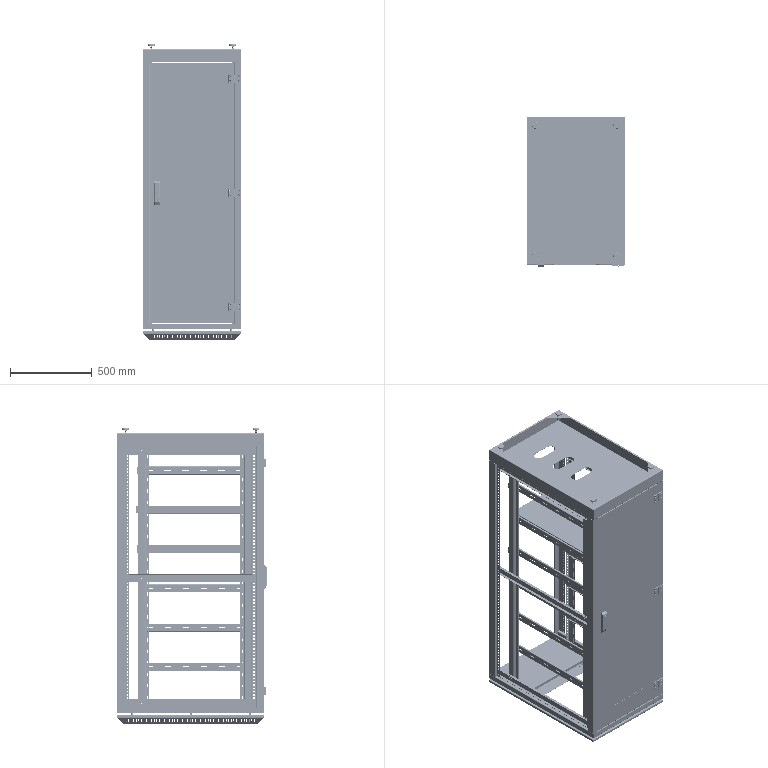Assembly | SolidWorks | mm | 69 component files | 69 solids | 8213 faces | box 600 x 916 x 1803.5 mm | volume 13058745 mm3 | plane 5185 | cylinder 2836 | spline 140 | cone 52 | commonest cylinder face diameters 3 x780 6 x617 5 x588 7 x278 12 x200 2 x165 10 x51 6.8 x40
Bill of materials:
ChassisWheel | 4 |  | Screw-like part: a large, flat, disc-shaped head with chamfered edges on a shorter, smaller-diameter shank that is threaded along most of its length.
Column | 3 |  | Long, slender bent sheet profile whose cross-section has several right-angle bends with rounded corners, forming a stepped, offset channel shape. A row of small perforations runs along its length.
Drawer | 1 |  | Shallow rectangular tray or cover panel: a flat face with short flanges folded down on all four edges.
Handle | 1 |  | Long bent sheet profile: a vertical wall, a flat top, an angled sloping section, and a short downturned lip, all with rounded bends.
828LockHead | 1 |  | Compact multi-feature body that looks like a latch or handle mechanism: an elongated front housing with a recessed face, a stepped rear body, a rectangular window, and a pin with a flanged head sticking out sideways.
LockRod | 2 |  | Pin with a flat tab: a flat, rounded-end tab with two through holes on top of a cylindrical rod with a conical tip.
LowerPullRod | 1 |  | Narrow flat strip with two joggle (offset) bends, giving a stepped profile, and two round holes near its rounded upper end.
UpperPullRod | 1 |  | Narrow flat strip with a single joggle bend: a long plain upper section and an offset lower section with a rounded end and two round holes.
BentPlate | 2 |  | Very long, slender U-channel with rounded bends and small holes spaced along its length.
GlassDoor | 1 |  | Thin flat rectangular frame panel with a large rounded-rectangle central cutout, two small rectangular cutouts in one side member, and small holes along the opposite edge.
ShortBentPlate_2 | 2 |  | Long bent sheet bracket with a stepped Z/hat-like section: a vertical web with three obround slots, a bottom flange, and an offset top flange that is shorter than the web.
ShortBentPlate | 2 |  | Straight C-channel with rounded bends and three small round holes in the web.
TemperedGlass5mm | 1 |  | Thin, plain rectangular flat plate, long and narrow, with no visible holes or cutouts.
GussetPlate | 4 |  | Thin flat plate shaped as a right-angle triangle with two equal legs and one circular through-hole near the right-angle corner.
Nut | 4 |  | Hexagonal prism with a central bore that has internal thread grooves (nut-like). One end has curved chamfered edges on the corners.
HexRod | 6 |  | Long, slender hexagonal bar with chamfered end corners and a threaded-looking axial hole at the visible end (standoff-like).
InnerColumn | 4 |  | Long formed sheet-metal profile with a stepped, multi-bend cross-section (a flange, a step, a long web and a return flange) with rounded bends, perforated along its length with regularly spaced slots and holes.
LeftColumn | 1 |  | Long formed sheet-metal profile with a complex stepped cross-section (outer flange, step, deep U-shaped section and opposite flange), rounded bends, small holes along one flange and notched ends.
LowerSeat | 1 |  | Shallow rectangular tray: a flat base with four upturned perimeter walls, three parallel obround slots in the base and small holes near the side edges.
OuterDoorHinge3 | 3 |  | Hinge-leaf-shaped plate: a flat rectangular leaf with two countersunk through-holes, an angled edge on one side, and three cylindrical knuckles with an axial bore along the opposite edge.
OuterHinge4 | 3 |  | Hinge-leaf-shaped plate: a flat rectangular leaf with two countersunk through-holes, an angled edge on one side, and two cylindrical knuckles with an axial bore along the opposite edge.
RailMountingBeam | 12 |  | Long, slender formed sheet-metal bracket/rail: a narrow web with six evenly spaced elongated slots, edge flanges, and a bent end tab at each end with two obround slots.
SideFixingBeam | 6 |  | Long straight bar with a rectangular, round-cornered cross-section (likely formed sheet), with one elongated slot near each end on one face and one small round hole near each end on an adjacent face.
TopCover | 1 |  | Rectangular sheet-metal panel/frame with a large rectangular cutout, inclined perimeter flanges with rows of narrow ventilation-style slots, and several small holes in the flat area.
UpperSeat2 | 1 |  | Thin, flat, U-shaped (forked) plate that looks like formed sheet metal. A solid rectangular region joins two long parallel legs, with a large rectangular open slot between them. Shallow flanges are bent down along the outer edges, and the face has small round through-holes.
UpperSill | 1 |  | Long, narrow, open-bottomed channel that looks like formed sheet metal. It has a flat top web and bent side walls with return lips at the bottom. One end is closed by a flange with a row of five evenly spaced round holes.
Mates:
1. coincident | LowerSeat-1 face at (-487.577, 386.781, 78) dir (1, 0, 0) | GussetPlateAssembly-1/GussetPlate-1 face at (-487.577, 276.923, 78) dir (-1, 0, 0)
2. coincident | LowerSeat-1 face at (98.282, 376.923, 78) dir (0, -1, 0) | GussetPlateAssembly-1/GussetPlate-1 face at (-487.577, 376.923, 78) dir (0, 1, 0)
3. coincident | LowerSeat-1 face at (-497.435, 386.923, 78) dir (0, 0, 1) | GussetPlateAssembly-1/GussetPlate-1 face at (-387.577, 376.923, 78) dir (0, 0, 1)
4. coincident | LowerSeat-1 face at (98.282, 376.923, 78) dir (0, -1, 0) | GussetPlateAssembly-2/GussetPlate-1 face at (-11.577, 376.923, 78) dir (0, 1, 0)
5. coincident | LowerSeat-1 face at (88.423, -508.936, 78) dir (-1, 0, 0) | GussetPlateAssembly-2/GussetPlate-1 face at (88.423, 376.923, 78) dir (1, 0, 0)
6. coincident | LowerSeat-1 face at (-497.435, 386.923, 78) dir (0, 0, 1) | GussetPlateAssembly-2/GussetPlate-1 face at (88.423, 276.923, 78) dir (0, 0, 1)
7. coincident | LowerSeat-1 face at (-497.435, -499.077, 78) dir (0, 1, 0) | GussetPlateAssembly-4/GussetPlate-1 face at (88.423, -499.077, 78) dir (0, -1, 0)
8. coincident | LowerSeat-1 face at (88.423, -508.936, 78) dir (-1, 0, 0) | GussetPlateAssembly-4/GussetPlate-1 face at (88.423, -399.077, 78) dir (1, 0, 0)
9. coincident | LowerSeat-1 face at (98.423, 386.781, 78) dir (0, 0, 1) | GussetPlateAssembly-4/GussetPlate-1 face at (-11.577, -499.077, 78) dir (0, 0, 1)
10. coincident | LowerSeat-1 face at (-487.577, 386.781, 78) dir (1, 0, 0) | GussetPlateAssembly-3/GussetPlate-1 face at (-487.577, -499.077, 78) dir (-1, 0, 0)
11. coincident | LowerSeat-1 face at (-497.435, -499.077, 78) dir (0, 1, 0) | GussetPlateAssembly-3/GussetPlate-1 face at (-387.577, -499.077, 78) dir (0, -1, 0)
12. coincident | LowerSeat-1 face at (98.282, -509.077, 78) dir (0, 0, 1) | GussetPlateAssembly-3/GussetPlate-1 face at (-487.577, -399.077, 78) dir (0, 0, 1)
13. coincident | LowerSeat-1 face at (-499.577, -511.077, 0) dir (-1, 0, 0) | Column-2 face at (-499.577, -461.077, -2) dir (-1, 0, 0)
14. coincident | LowerSeat-1 face at (-499.577, -511.077, 78) dir (0, -1, 0) | Column-2 face at (-499.577, -511.077, -2) dir (0, -1, 0)
15. coincident | LowerSeat-1 face at (100.423, -511.077, -2) dir (0, 0, -1) | Column-2 face at (-496.577, -509.077, -2) dir (0, 0, 1)
16. coincident | LowerSeat-1 face at (100.423, 388.923, 78) dir (0, 1, 0) | Column-3 face at (-499.577, 388.923, -1597) dir (0, 1, 0)
17. coincident | LowerSeat-1 face at (-499.577, -511.077, 0) dir (-1, 0, 0) | Column-3 face at (-499.577, 338.923, -1597) dir (-1, 0, 0)
18. coincident | LowerSeat-1 face at (100.423, -511.077, -2) dir (0, 0, -1) | Column-3 face at (-496.577, 340.923, -2) dir (0, 0, 1)
19. coincident | LowerSeat-1 face at (100.423, 388.923, 78) dir (0, 1, 0) | Column-4 face at (100.423, 388.923, -2) dir (0, 1, 0)
20. coincident | LowerSeat-1 face at (100.423, -511.077, 78) dir (1, 0, 0) | Column-4 face at (100.423, 338.923, -2) dir (1, 0, 0)
21. coincident | LowerSeat-1 face at (100.423, -511.077, -2) dir (0, 0, -1) | Column-4 face at (62.423, 385.923, -2) dir (0, 0, 1)
22. coincident | Column-3 face at (-499.577, 388.923, -1597) dir (0, 1, 0) | UpperSeatAssembly-1/UpperSeat2-1 face at (100.423, 388.923, -1599) dir (0, 1, 0)
23. coincident | Column-3 face at (-499.577, 338.923, -1597) dir (-1, 0, 0) | UpperSeatAssembly-1/UpperSeat2-1 face at (-499.577, 388.923, -1599) dir (-1, 0, 0)
24. coincident | Column-3 face at (-496.577, 386.923, -1597) dir (0, 0, -1) | UpperSeatAssembly-1/UpperSeat2-1 face at (100.423, -511.077, -1597) dir (0, 0, 1)
25. coincident | LowerSeat-1 face at (100.423, -511.077, -2) dir (0, 0, -1) | SideFixingBeam-1 face at (-479.577, -488.077, -2) dir (0, 0, 1)
26. coincident | Column-3 face at (-479.577, 315.923, -1597) dir (1, 0, 0) | SideFixingBeam-1 face at (-479.577, 361.923, -2) dir (-1, 0, 0)
27. coincident | Column-3 face at (-459.577, 361.923, -1597) dir (0, -1, 0) | SideFixingBeam-1 face at (-479.577, 361.923, -2) dir (0, 1, 0)
28. coincident | LowerSeat-1 face at (100.423, -511.077, -2) dir (0, 0, -1) | SideFixingBeam-2 face at (80.423, 361.923, -2) dir (0, 0, 1)
29. coincident | Column-4 face at (62.423, 388.923, -2) dir (1, 0, 0) | SideFixingBeam-2 face at (62.423, 361.923, -2) dir (-1, 0, 0)
30. coincident | Column-4 face at (60.423, 361.923, -2) dir (0, -1, 0) | SideFixingBeam-2 face at (80.423, 361.923, -52) dir (0, 1, 0)
31. coincident | Column-4 face at (62.423, 388.923, -2) dir (1, 0, 0) | SideFixingBeam-3 face at (62.423, 361.923, -1547) dir (-1, 0, 0)
32. coincident | UpperSeatAssembly-1/UpperSeat2-1 face at (100.423, -511.077, -1597) dir (0, 0, 1) | SideFixingBeam-3 face at (80.423, -488.077, -1597) dir (0, 0, -1)
33. coincident | Column-4 face at (60.423, 361.923, -2) dir (0, -1, 0) | SideFixingBeam-3 face at (80.423, 361.923, -1597) dir (0, 1, 0)
34. coincident | Column-3 face at (-461.577, 388.923, -1597) dir (-1, 0, 0) | SideFixingBeam-5 face at (-461.577, 361.923, -1597) dir (1, 0, 0)
35. coincident | UpperSeatAssembly-1/UpperSeat2-1 face at (100.423, -511.077, -1597) dir (0, 0, 1) | SideFixingBeam-5 face at (-479.577, 361.923, -1597) dir (0, 0, -1)
36. coincident | Column-3 face at (-459.577, 361.923, -1597) dir (0, -1, 0) | SideFixingBeam-5 face at (-479.577, 361.923, -1547) dir (0, 1, 0)
37. coincident | Column-4 face at (60.423, 361.923, -2) dir (0, -1, 0) | SideFixingBeam-6 face at (80.423, 361.923, -832) dir (0, 1, 0)
38. coincident | Column-3 face at (-461.577, 388.923, -1597) dir (-1, 0, 0) | SideFixingBeam-7 face at (-461.577, 361.923, -832) dir (1, 0, 0)
39. coincident | Column-3 face at (-459.577, 361.923, -1597) dir (0, -1, 0) | SideFixingBeam-7 face at (-479.577, 361.923, -782) dir (0, 1, 0)
40. coincident | SideFixingBeam-1 face at (-461.577, 361.923, -52) dir (1, 0, 0) | InnerColumn-1 face at (-461.577, -388.077, -4.5) dir (-1, 0, 0)
41. distance | InnerColumn-1 face at (-461.577, -433.077, -4.5) dir (0, -1, 0) | LowerSeat-1 face at (-499.577, -511.077, 78) dir (0, -1, 0)
42. coincident | SideFixingBeam-2 face at (62.423, 361.923, -2) dir (-1, 0, 0) | InnerColumn-2 face at (62.423, -388.077, -1594.5) dir (1, 0, 0)
43. distance | InnerColumn-2 face at (62.423, -433.077, -1594.5) dir (0, -1, 0) | LowerSeat-1 face at (-499.577, -511.077, 78) dir (0, -1, 0)
44. distance | LowerSeat-1 face at (100.423, -511.077, -2) dir (0, 0, -1) | InnerColumn-1 face at (-458.577, -431.077, -4.5) dir (0, 0, 1)
45. distance | LowerSeat-1 face at (100.423, -511.077, -2) dir (0, 0, -1) | InnerColumn-2 face at (59.423, -390.077, -4.5) dir (0, 0, 1)
46. coincident | SideFixingBeam-2 face at (62.423, 361.923, -2) dir (-1, 0, 0) | InnerColumn-3 face at (62.423, 215.923, -4.5) dir (1, 0, 0)
47. distance | InnerColumn-3 face at (59.423, 258.923, -4.5) dir (0, 0, 1) | LowerSeat-1 face at (100.423, -511.077, -2) dir (0, 0, -1)
48. coincident | SideFixingBeam-1 face at (-461.577, 361.923, -52) dir (1, 0, 0) | InnerColumn-4 face at (-461.577, 215.923, -1594.5) dir (-1, 0, 0)
49. distance | LowerSeat-1 face at (100.423, -511.077, -2) dir (0, 0, -1) | InnerColumn-4 face at (-458.577, 217.923, -4.5) dir (0, 0, 1)
50. distance | InnerColumn-3 face at (62.423, 260.923, -4.5) dir (0, 1, 0) | Column-4 face at (100.423, 388.923, -2) dir (0, 1, 0)
51. distance | InnerColumn-4 face at (-461.577, 260.923, -1594.5) dir (0, 1, 0) | Column-3 face at (-499.577, 388.923, -1597) dir (0, 1, 0)
52. distance | LowerSeat-1 face at (100.423, -511.077, -2) dir (0, 0, -1) | SideFixingBeam-7 face at (-479.577, -488.077, -782) dir (0, 0, 1)
53. distance | SideFixingBeam-6 face at (80.423, 361.923, -782) dir (0, 0, 1) | LowerSeat-1 face at (100.423, -511.077, -2) dir (0, 0, -1)
54. coincident | InnerColumn-2 face at (62.423, -433.077, -1594.5) dir (0, -1, 0) | RailMountingBeam-1 face at (57.423, -433.077, -127) dir (0, 1, 0)
55. distance | RailMountingBeam-1 face at (57.423, -435.077, -127) dir (1, 0, 0) | InnerColumn-2 face at (62.423, -388.077, -1594.5) dir (1, 0, 0)
56. coincident | InnerColumn-1 face at (-461.577, -433.077, -4.5) dir (0, -1, 0) | RailMountingBeam-2 face at (-456.577, -433.077, -171) dir (0, 1, 0)
57. distance | InnerColumn-1 face at (-461.577, -388.077, -4.5) dir (-1, 0, 0) | RailMountingBeam-2 face at (-456.577, -435.077, -171) dir (-1, 0, 0)
58. distance | LowerSeat-1 face at (100.423, -511.077, -2) dir (0, 0, -1) | RailMountingBeam-2 face at (-431.577, -435.077, -124) dir (0, 0, 1)
59. distance | LowerSeat-1 face at (100.423, -511.077, -2) dir (0, 0, -1) | RailMountingBeam-1 face at (32.423, 264.923, -124) dir (0, 0, 1)
60. coincident | InnerColumn-4 face at (-461.577, 260.923, -1594.5) dir (0, 1, 0) | RailMountingBeam-3 face at (-456.577, 260.923, -367) dir (0, -1, 0)
61. distance | RailMountingBeam-3 face at (-456.577, 262.923, -367) dir (-1, 0, 0) | InnerColumn-4 face at (-461.577, 215.923, -1594.5) dir (-1, 0, 0)
62. distance | RailMountingBeam-2 face at (-431.577, 264.923, -174) dir (0, 0, -1) | RailMountingBeam-3 face at (-431.577, -437.077, -364) dir (0, 0, 1)
63. coincident | InnerColumn-2 face at (62.423, -433.077, -1594.5) dir (0, -1, 0) | RailMountingBeam-4 face at (57.423, -433.077, -367) dir (0, 1, 0)
64. distance | RailMountingBeam-4 face at (57.423, -435.077, -367) dir (1, 0, 0) | InnerColumn-2 face at (62.423, -388.077, -1594.5) dir (1, 0, 0)
65. distance | RailMountingBeam-1 face at (32.423, -435.077, -174) dir (0, 0, -1) | RailMountingBeam-4 face at (32.423, 264.923, -364) dir (0, 0, 1)
66. coincident | InnerColumn-2 face at (62.423, -433.077, -1594.5) dir (0, -1, 0) | RailMountingBeam-5 face at (57.423, -433.077, -607) dir (0, 1, 0)
67. distance | RailMountingBeam-5 face at (57.423, -435.077, -607) dir (1, 0, 0) | InnerColumn-2 face at (62.423, -388.077, -1594.5) dir (1, 0, 0)
68. distance | RailMountingBeam-4 face at (32.423, -435.077, -414) dir (0, 0, -1) | RailMountingBeam-5 face at (32.423, 264.923, -604) dir (0, 0, 1)
69. coincident | InnerColumn-1 face at (-461.577, -433.077, -4.5) dir (0, -1, 0) | RailMountingBeam-6 face at (-456.577, -433.077, -651) dir (0, 1, 0)
70. distance | RailMountingBeam-3 face at (-431.577, 262.923, -414) dir (0, 0, -1) | RailMountingBeam-6 face at (-431.577, -435.077, -604) dir (0, 0, 1)
71. distance | RailMountingBeam-6 face at (-456.577, -435.077, -651) dir (-1, 0, 0) | InnerColumn-1 face at (-461.577, -388.077, -4.5) dir (-1, 0, 0)
72. coincident | InnerColumn-3 face at (62.423, 260.923, -4.5) dir (0, 1, 0) | RailMountingBeam-7 face at (57.423, 260.923, -891) dir (0, -1, 0)
73. distance | RailMountingBeam-7 face at (57.423, 262.923, -891) dir (1, 0, 0) | InnerColumn-3 face at (62.423, 215.923, -4.5) dir (1, 0, 0)
74. distance | RailMountingBeam-5 face at (32.423, -435.077, -654) dir (0, 0, -1) | RailMountingBeam-7 face at (32.423, 262.923, -844) dir (0, 0, 1)
75. coincident | InnerColumn-4 face at (-461.577, 260.923, -1594.5) dir (0, 1, 0) | RailMountingBeam-8 face at (-456.577, 260.923, -847) dir (0, -1, 0)
76. distance | RailMountingBeam-8 face at (-456.577, 262.923, -847) dir (-1, 0, 0) | InnerColumn-4 face at (-461.577, 215.923, -1594.5) dir (-1, 0, 0)
77. distance | RailMountingBeam-6 face at (-431.577, 264.923, -654) dir (0, 0, -1) | RailMountingBeam-8 face at (-431.577, -437.077, -844) dir (0, 0, 1)
78. coincident | InnerColumn-4 face at (-461.577, 260.923, -1594.5) dir (0, 1, 0) | RailMountingBeam-9 face at (-456.577, 260.923, -1087) dir (0, -1, 0)
79. distance | InnerColumn-4 face at (-461.577, 215.923, -1594.5) dir (-1, 0, 0) | RailMountingBeam-9 face at (-456.577, 262.923, -1087) dir (-1, 0, 0)
80. distance | RailMountingBeam-8 face at (-431.577, 262.923, -894) dir (0, 0, -1) | RailMountingBeam-9 face at (-431.577, -437.077, -1084) dir (0, 0, 1)
81. distance | RailMountingBeam-10 face at (57.423, 262.923, -1131) dir (1, 0, 0) | InnerColumn-3 face at (62.423, 215.923, -4.5) dir (1, 0, 0)
82. coincident | InnerColumn-3 face at (62.423, 260.923, -4.5) dir (0, 1, 0) | RailMountingBeam-10 face at (57.423, 260.923, -1131) dir (0, -1, 0)
83. distance | RailMountingBeam-7 face at (32.423, -437.077, -894) dir (0, 0, -1) | RailMountingBeam-10 face at (32.423, 262.923, -1084) dir (0, 0, 1)
84. coincident | InnerColumn-4 face at (-461.577, 260.923, -1594.5) dir (0, 1, 0) | RailMountingBeam-11 face at (-456.577, 260.923, -1327) dir (0, -1, 0)
85. distance | RailMountingBeam-11 face at (-456.577, 262.923, -1327) dir (-1, 0, 0) | InnerColumn-4 face at (-461.577, 215.923, -1594.5) dir (-1, 0, 0)
86. distance | RailMountingBeam-9 face at (-431.577, 262.923, -1134) dir (0, 0, -1) | RailMountingBeam-11 face at (-431.577, -437.077, -1324) dir (0, 0, 1)
87. coincident | InnerColumn-3 face at (62.423, 260.923, -4.5) dir (0, 1, 0) | RailMountingBeam-12 face at (57.423, 260.923, -1371) dir (0, -1, 0)
88. distance | RailMountingBeam-12 face at (57.423, 262.923, -1371) dir (1, 0, 0) | InnerColumn-3 face at (62.423, 215.923, -4.5) dir (1, 0, 0)
89. distance | RailMountingBeam-10 face at (32.423, -437.077, -1134) dir (0, 0, -1) | RailMountingBeam-12 face at (32.423, 262.923, -1324) dir (0, 0, 1)
90. concentric | UpperSeatAssembly-1/UpperSeat2-1 face at (38.423, 298.923, -1599) dir (0, 0, 1) r 3.5 | HexRod-1 face at (38.423, 298.923, -1619) dir (0, 0, 1) r 3
91. coincident | UpperSeatAssembly-1/UpperSeat2-1 face at (100.423, -511.077, -1599) dir (0, 0, -1) | HexRod-1 face at (42.64, 302.866, -1599) dir (0, 0, 1)
92. concentric | UpperSeatAssembly-1/UpperSeat2-1 face at (38.423, -61.077, -1599) dir (0, 0, 1) r 3.5 | HexRod-3 face at (38.423, -61.077, -1619) dir (0, 0, 1) r 3
93. coincident | UpperSeatAssembly-1/UpperSeat2-1 face at (100.423, -511.077, -1599) dir (0, 0, -1) | HexRod-3 face at (43.423, -58.191, -1599) dir (0, 0, 1)
94. concentric | UpperSeatAssembly-1/UpperSeat2-1 face at (38.423, -421.077, -1599) dir (0, 0, 1) r 3.5 | HexRod-4 face at (38.423, -421.077, -1619) dir (0, 0, 1) r 3
95. coincident | UpperSeatAssembly-1/UpperSeat2-1 face at (100.423, -511.077, -1599) dir (0, 0, -1) | HexRod-4 face at (43.423, -418.191, -1599) dir (0, 0, 1)
96. concentric | UpperSeatAssembly-1/UpperSeat2-1 face at (-437.577, 298.923, -1599) dir (0, 0, 1) r 3.5 | HexRod-5 face at (-437.577, 298.923, -1619) dir (0, 0, 1) r 3
97. coincident | UpperSeatAssembly-1/UpperSeat2-1 face at (100.423, -511.077, -1599) dir (0, 0, -1) | HexRod-5 face at (-431.803, 298.923, -1599) dir (0, 0, 1)
98. concentric | UpperSeatAssembly-1/UpperSeat2-1 face at (-437.577, -61.077, -1599) dir (0, 0, 1) r 3.5 | HexRod-7 face at (-437.577, -61.077, -1619) dir (0, 0, 1) r 3
99. coincident | UpperSeatAssembly-1/UpperSeat2-1 face at (100.423, -511.077, -1599) dir (0, 0, -1) | HexRod-7 face at (-432.577, -58.191, -1599) dir (0, 0, 1)
100. concentric | UpperSeatAssembly-1/UpperSeat2-1 face at (-437.577, -421.077, -1599) dir (0, 0, 1) r 3.5 | HexRod-8 face at (-437.577, -421.077, -1619) dir (0, 0, 1) r 3
101. coincident | UpperSeatAssembly-1/UpperSeat2-1 face at (100.423, -511.077, -1599) dir (0, 0, -1) | HexRod-8 face at (-432.577, -418.191, -1599) dir (0, 0, 1)
102. coincident | UpperSeatAssembly-1/UpperSeat2-1 face at (-499.577, 388.923, -1599) dir (-1, 0, 0) | TopCover-1 face at (-499.577, -4622.172, -1658.645) dir (-1, 0, 0)
103. coincident | UpperSeatAssembly-1/UpperSill-1 face at (30.423, -511.077, -1632) dir (0, -1, 0) | TopCover-1 face at (4211.519, -511.077, -1658.645) dir (0, -1, 0)
104. coincident | HexRod-8 face at (-432.577, -418.191, -1694) dir (0, 0, -1) | TopCover-1 face at (65.069, -475.722, -1694) dir (0, 0, 1)
105. concentric | GussetPlateAssembly-3/Nut-1 face at (-447.577, -459.077, 76) dir (0, 0, -1) r 6 | ChassisWheel-1 face at (-447.577, -459.077, 68) dir (0, 0, 1) r 6
106. distance | GussetPlateAssembly-3/GussetPlate-1 face at (-487.577, -399.077, 78) dir (0, 0, 1) | ChassisWheel-1 face at (-447.577, -459.077, 98) dir (0, 0, -1)
107. concentric | GussetPlateAssembly-4/Nut-1 face at (48.423, -459.077, 76) dir (0, 0, -1) r 6 | ChassisWheel-2 face at (48.423, -459.077, 68) dir (0, 0, 1) r 6
108. distance | GussetPlateAssembly-4/GussetPlate-1 face at (-11.577, -499.077, 78) dir (0, 0, 1) | ChassisWheel-2 face at (48.423, -459.077, 98) dir (0, 0, -1)
109. concentric | GussetPlateAssembly-1/Nut-1 face at (-447.577, 336.923, 76) dir (0, 0, -1) r 6 | ChassisWheel-3 face at (-447.577, 336.923, 68) dir (0, 0, 1) r 6
110. concentric | GussetPlateAssembly-1/Nut-1 face at (-447.577, 336.923, 76) dir (0, 0, -1) r 6 | ChassisWheel-3 face at (-447.577, 336.923, 68) dir (0, 0, 1) r 6
111. distance | GussetPlateAssembly-1/GussetPlate-1 face at (-387.577, 376.923, 78) dir (0, 0, 1) | ChassisWheel-3 face at (-447.577, 336.923, 98) dir (0, 0, -1)
112. concentric | GussetPlateAssembly-2/Nut-1 face at (48.423, 336.923, 76) dir (0, 0, -1) r 6 | ChassisWheel-4 face at (48.423, 336.923, 68) dir (0, 0, 1) r 6
113. distance | GussetPlateAssembly-2/GussetPlate-1 face at (88.423, 276.923, 78) dir (0, 0, 1) | ChassisWheel-4 face at (48.423, 336.923, 98) dir (0, 0, -1)
114. coincident | UpperSeatAssembly-1/UpperSeat2-1 face at (30.423, -511.077, -1599) dir (0, -1, 0) | LeftColumn-1 face at (100.423, -511.077, -1597) dir (0, -1, 0)
115. coincident | UpperSeatAssembly-1/UpperSeat2-1 face at (100.423, -511.077, -1599) dir (1, 0, 0) | LeftColumn-1 face at (100.423, -461.077, -1597) dir (1, 0, 0)
116. coincident | UpperSeatAssembly-1/UpperSeat2-1 face at (100.423, -511.077, -1597) dir (0, 0, 1) | LeftColumn-1 face at (97.423, -509.077, -1597) dir (0, 0, -1)
117. coincident | Column-4 face at (60.423, 361.923, -2) dir (0, -1, 0) | SideFixingBeam-6 face at (80.423, 361.923, -832) dir (0, 1, 0)
118. tangent | Column-4 face at (59.423, 364.923, -2) dir (0, 0, -1) r 3 | SideFixingBeam-6 face at (62.423, 361.923, -782) dir (-1, 0, 0)
119. concentric | LeftColumn-1 face at (85.923, -509.077, -1512) dir (0, -1, 0) r 3 | OuterDoorHingeAssembly1-1/OuterHinge4-1 face at (85.923, -507.077, -1512) dir (0, -1, 0) r 3
120. concentric | LeftColumn-1 face at (85.923, -509.077, -1482) dir (0, -1, 0) r 3 | OuterDoorHingeAssembly1-1/OuterHinge4-1 face at (85.923, -507.077, -1482) dir (0, -1, 0) r 3
121. coincident | LeftColumn-1 face at (100.423, -511.077, -1597) dir (0, -1, 0) | OuterDoorHingeAssembly1-1/OuterHinge4-1 face at (96.923, -511.077, -1472) dir (0, 1, 0)
122. concentric | LeftColumn-1 face at (85.923, -509.077, -814.5) dir (0, -1, 0) r 3 | OuterDoorHingeAssembly1-2/OuterHinge4-1 face at (85.923, -507.077, -814.5) dir (0, -1, 0) r 3
123. concentric | LeftColumn-1 face at (85.923, -509.077, -784.5) dir (0, -1, 0) r 3 | OuterDoorHingeAssembly1-2/OuterHinge4-1 face at (85.923, -507.077, -784.5) dir (0, -1, 0) r 3
124. coincident | LeftColumn-1 face at (100.423, -511.077, -1597) dir (0, -1, 0) | OuterDoorHingeAssembly1-2/OuterHinge4-1 face at (96.923, -511.077, -774.5) dir (0, 1, 0)
125. concentric | LeftColumn-1 face at (85.923, -509.077, -117) dir (0, -1, 0) r 3 | OuterDoorHingeAssembly1-3/OuterHinge4-1 face at (85.923, -507.077, -117) dir (0, -1, 0) r 3
126. concentric | LeftColumn-1 face at (85.923, -509.077, -87) dir (0, -1, 0) r 3 | OuterDoorHingeAssembly1-3/OuterHinge4-1 face at (85.923, -507.077, -87) dir (0, -1, 0) r 3
127. coincident | LeftColumn-1 face at (100.423, -511.077, -1597) dir (0, -1, 0) | OuterDoorHingeAssembly1-3/OuterHinge4-1 face at (96.923, -511.077, -77) dir (0, 1, 0)
128. distance | GlassDoorAssembly-1/GlassDoor-1 face at (-457.577, -486.077, -1595) dir (0, 0, -1) | UpperSeatAssembly-1/UpperSill-1 face at (30.423, -411.077, -1597) dir (0, 0, 1)
129. distance | GlassDoorAssembly-1/GlassDoor-1 face at (58.423, -486.077, -4) dir (1, 0, 0) | LeftColumn-1 face at (60.423, -511.077, -1597) dir (-1, 0, 0)
130. coincident | LeftColumn-1 face at (100.423, -511.077, -1597) dir (0, -1, 0) | GlassDoorAssembly-1/GlassDoor-1 face at (58.423, -511.077, -1595) dir (0, -1, 0)
131. distance | DrawerAssembly-1/Drawer-1 face at (12.923, 272.545, -409) dir (1, 0, 0) | RailMountingBeam-4 face at (32.423, -435.077, -364) dir (-1, 0, 0)
132. distance | DrawerAssembly-1/Drawer-1 face at (-412.077, -427.455, -369) dir (0, 0, 1) | RailMountingBeam-4 face at (32.423, 264.923, -366) dir (0, 0, -1)
133. coincident | Drawer-1 face at (-377.093, -394.828, 40) dir (0, -1, 0) | Handle-1 face at (-392.093, -394.828, 44.3) dir (0, 1, 0)
134. distance | Drawer-1 face at (-377.093, 305.172, 40) dir (-1, 0, 0) | Handle-1 face at (-392.093, -440.828, 14.918) dir (-1, 0, 0)
135. distance | Drawer-1 face at (47.907, -394.828, 0) dir (0, 0, -1) | Handle-1 face at (-392.093, -396.828, 2.3) dir (0, 0, -1)
136. coincident | GlassDoor-1 face at (586.595, -219.27, 2) dir (0, 0, 1) | BentPlate-1 face at (-932.405, -122.27, 2) dir (0, 0, -1)
137. distance | BentPlate-1 face at (-932.405, -122.27, 2) dir (0, 1, 0) | GlassDoor-1 face at (441.595, -99.27, 2) dir (0, 1, 0)
138. distance | GlassDoor-1 face at (-884.405, -74.27, 2) dir (1, 0, 0) | BentPlate-1 face at (-932.405, -122.27, 16.5) dir (-1, 0, 0)
139. coincident | GlassDoor-1 face at (586.595, -219.27, 2) dir (0, 0, 1) | BentPlate-2 face at (-932.405, 224.73, 2) dir (0, 0, -1)
140. distance | BentPlate-2 face at (512.595, 199.73, 2) dir (0, -1, 0) | GlassDoor-1 face at (441.595, 176.73, 2) dir (0, -1, 0)
141. distance | BentPlate-2 face at (-932.405, 199.73, 2) dir (-1, 0, 0) | GlassDoor-1 face at (-884.405, -74.27, 2) dir (1, 0, 0)
142. coincident | GlassDoor-1 face at (586.595, -219.27, 2) dir (0, 0, 1) | ShortBentPlate-5 face at (512.595, 199.73, 2) dir (0, 0, -1)
143. coincident | BentPlate-2 face at (512.595, 199.73, 16.5) dir (1, 0, 0) | ShortBentPlate-5 face at (512.595, 199.73, 2) dir (1, 0, 0)
144. coincident | BentPlate-2 face at (512.595, 199.73, 2) dir (0, -1, 0) | ShortBentPlate-5 face at (512.595, 199.73, 16.5) dir (0, 1, 0)
145. coincident | GlassDoor-1 face at (586.595, -219.27, 2) dir (0, 0, 1) | ShortBentPlate-6 face at (-907.405, 197.73, 2) dir (0, 0, -1)
146. coincident | BentPlate-1 face at (-932.405, -122.27, 16.5) dir (-1, 0, 0) | ShortBentPlate-6 face at (-932.405, -122.27, 2) dir (-1, 0, 0)
147. coincident | BentPlate-1 face at (-932.405, -122.27, 2) dir (0, 1, 0) | ShortBentPlate-6 face at (-932.405, -122.27, 16.5) dir (0, -1, 0)
148. coincident | GlassDoor-1 face at (586.595, -219.27, 2) dir (0, 0, 1) | ShortBentPlate_2-1 face at (520.095, 191.23, 2) dir (0, 0, -1)
149. distance | ShortBentPlate_2-1 face at (518.595, 191.23, 2) dir (-1, 0, 0) | ShortBentPlate-5 face at (512.595, 199.73, 2) dir (1, 0, 0)
150. coincident | GlassDoor-1 face at (586.595, -219.27, 2) dir (0, 0, 1) | ShortBentPlate_2-2 face at (-939.905, -113.77, 2) dir (0, 0, -1)
151. distance | ShortBentPlate-6 face at (-907.405, 197.73, 2) dir (1, 0, 0) | ShortBentPlate_2-2 face at (-901.405, -113.77, 18.5) dir (-1, 0, 0)
152. coincident | GlassDoor-1 face at (586.595, -219.27, 2) dir (0, 0, 1) | TemperedGlass5mm-2 face at (482.595, -117.27, 2) dir (0, 0, -1)
153. distance | TemperedGlass5mm-2 face at (-902.405, -117.27, 2) dir (0, -1, 0) | BentPlate-1 face at (-932.405, -122.27, 2) dir (0, 1, 0)
154. distance | TemperedGlass5mm-2 face at (482.595, 192.73, 2) dir (1, 0, 0) | ShortBentPlate-5 face at (487.595, -120.27, 2) dir (-1, 0, 0)
155. coincident | GlassDoor-1 face at (586.595, -219.27, 0) dir (0, 0, -1) | 828LockAssembly-1/828LockHead-1 face at (-134.405, 269.23, 0) dir (0, 0, 1)
156. coincident | GlassDoor-1 face at (-150.405, 264.73, 2) dir (0, -1, 0) | 828LockAssembly-1/828LockHead-1 face at (-138.405, 264.73, 20) dir (0, 1, 0)
157. coincident | GlassDoor-1 face at (-234.405, 238.73, 2) dir (-1, 0, 0) | 828LockAssembly-1/828LockHead-1 face at (-234.405, 264.73, 17) dir (1, 0, 0)
158. coincident | 828LockHead-1 face at (-43.998, -17.233, 31) dir (-1, 0, 0) | UpperPullRod-1 face at (-43.998, -114.41, 31) dir (1, 0, 0)
159. coincident | 828LockHead-1 face at (-46.998, -17.233, 31) dir (0, 0, -1) | UpperPullRod-1 face at (-46.998, -17.41, 31) dir (0, 0, 1)
160. coincident | 828LockHead-1 face at (-25.998, -17.233, 31) dir (1, 0, 0) | LowerPullRod-1 face at (-25.998, -4.141, 31) dir (-1, 0, 0)
161. coincident | 828LockHead-1 face at (-25.998, -17.233, 31) dir (0, 0, -1) | LowerPullRod-1 face at (-22.998, -77.141, 31) dir (0, 0, 1)
162. concentric | UpperPullRod-1 face at (-33.392, -165.016, 24.5) dir (-1, 0, 0) r 3.25 | LockRod-1 face at (-33.392, -165.016, 24.5) dir (1, 0, 0) r 3.25
163. concentric | UpperPullRod-1 face at (-33.392, -140.016, 24.5) dir (-1, 0, 0) r 3.25 | LockRod-1 face at (-33.392, -140.016, 24.5) dir (1, 0, 0) r 3.25
164. coincident | UpperPullRod-1 face at (-33.392, -126.259, 31) dir (1, 0, 0) | LockRod-1 face at (-33.392, -132.016, 17) dir (-1, 0, 0)
165. concentric | LowerPullRod-1 face at (-28.263, 106.741, 24.5) dir (1, 0, 0) r 3.25 | LockRod-2 face at (-33.263, 106.741, 24.5) dir (1, 0, 0) r 3.25
166. concentric | LowerPullRod-1 face at (-28.263, 131.741, 24.5) dir (1, 0, 0) r 3.25 | LockRod-2 face at (-33.263, 131.741, 24.5) dir (1, 0, 0) r 3.25
167. coincident | LowerPullRod-1 face at (-28.263, 139.741, 18) dir (-1, 0, 0) | LockRod-2 face at (-28.263, 98.741, 32) dir (1, 0, 0)
168. concentric | GussetPlate-1 face at (-17.264, -13.154, -2) dir (0, 0, 1) r 7.5 | Nut-1 face at (-17.264, -13.154, 0) dir (0, 0, 1) r 6
169. coincident | GussetPlate-1 face at (42.736, -53.154, 0) dir (0, 0, 1) | Nut-1 face at (-4.57, -12.722, 0) dir (0, 0, -1)
170. concentric | OuterDoorHinge3-1 face at (12.913, 26.96, 1) dir (0, -1, 0) r 3 | OuterHinge4-1 face at (12.913, -43.04, 1) dir (0, 1, 0) r 3
171. coincident | OuterDoorHinge3-1 face at (7.913, 6.96, 9) dir (0, -1, 0) | OuterHinge4-1 face at (18.443, 6.96, 9) dir (0, 1, 0)
172. coincident | UpperSeat2-1 face at (67.734, -512.798, 0) dir (0, 0, 1) | UpperSill-1 face at (-2.266, -412.798, 0) dir (0, 0, 1)
173. coincident | UpperSeat2-1 face at (-532.266, -512.798, -2) dir (0, -1, 0) | UpperSill-1 face at (-2.266, -512.798, -35) dir (0, -1, 0)
174. coincident | UpperSeat2-1 face at (-462.266, -509.798, -2) dir (1, 0, 0) | UpperSill-1 face at (-462.266, -509.798, -20) dir (-1, 0, 0)